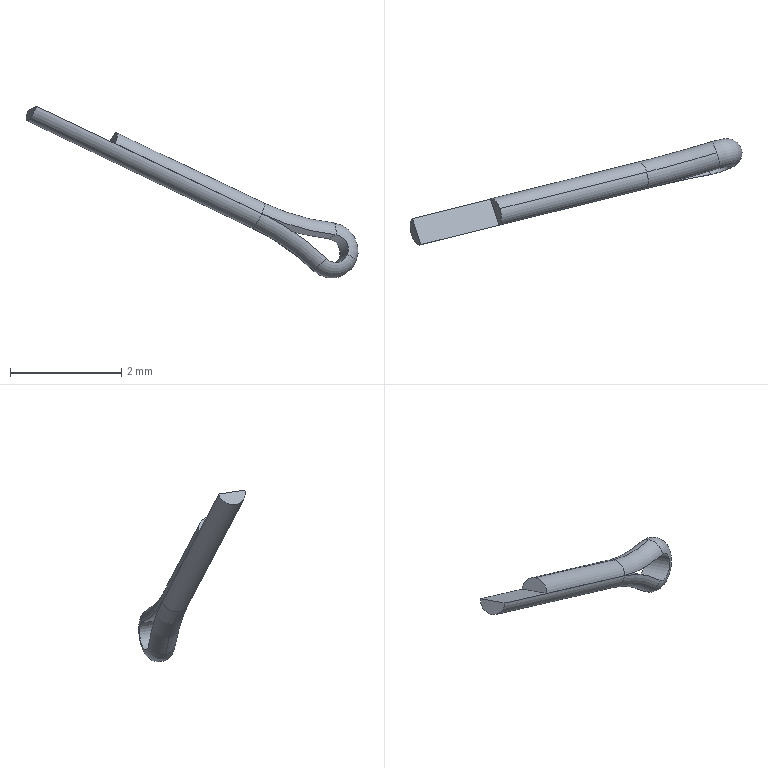Component | SolidWorks | split pins-2 | 1 solid | 16 faces | volume 1 mm3 | torus 6 | cylinder 6 | plane 4 | commonest cylinder face diameters 0.5 x4 8.75 x2
build123d program:
from build123d import *


with BuildPart() as part:
    # Body: sweep along a path in PathSke
    with BuildLine(Plane(origin=(1.208, 1.808, 0), x_dir=(0, 1, 0), z_dir=(0, 0, 1))) as body_path:
        Line((-1.558, -3.792), (-1.558, -0.792))
        ThreePointArc((-1.558, -0.792), (-1.502, -0.1139), (-1.335, 0.5458))
        ThreePointArc((-1.335, 0.5458), (-1.808, 1.208), (-2.281, 0.5458))
        ThreePointArc((-2.281, 0.5458), (-2.114, -0.1139), (-2.058, -0.792))
        Line((-2.058, -0.792), (-2.058, -5.392))
    # SectionSke → Body (sweep)
    with BuildSketch(Plane(origin=(5, 0.15, 0.15), x_dir=(0, 1, 0), z_dir=(1, 0, 0))):
        with BuildLine():
            Line((-0.15, -0.4), (-0.15, 0.1))
            ThreePointArc((-0.15, 0.1), (0.1, -0.15), (-0.15, -0.4))
        make_face()
    sweep(path=body_path.line)


solid = part.part

# Placed as in the assembly
solid = solid.moved(Location((-260.959, -17.55, 167.563), (-98.133, -17.491, -157.4)))
STEP:
#1=CARTESIAN_POINT('',(-10.34,-0.7059,6.639));
#2=VERTEX_POINT('',#1);
#3=CARTESIAN_POINT('',(-10.346,-0.699,6.629));
#4=VERTEX_POINT('',#3);
#5=CARTESIAN_POINT('',(-10.343,-0.7083,6.63));
#6=DIRECTION('',(-0.8805,-0.2203,0.4197));
#7=DIRECTION('',(0.3006,-0.9442,0.1349));
#8=AXIS2_PLACEMENT_3D('',#5,#6,#7);
#9=CIRCLE('',#8,0.009843);
#10=EDGE_CURVE('',#2,#4,#9,.T.);
#11=ORIENTED_EDGE('',*,*,#10,.F.);
#12=CARTESIAN_POINT('',(-10.29,-0.6921,6.625));
#13=VERTEX_POINT('',#12);
#14=CARTESIAN_POINT('',(-10.28,-0.6661,6.785));
#15=DIRECTION('',(0.3006,-0.9442,0.1349));
#16=DIRECTION('',(0.9529,0.3033,0.));
#17=AXIS2_PLACEMENT_3D('',#14,#15,#16);
#18=CIRCLE('',#17,0.1624);
#19=EDGE_CURVE('',#2,#13,#18,.T.);
#20=ORIENTED_EDGE('',*,*,#19,.T.);
#21=CARTESIAN_POINT('',(-10.294,-0.6844,6.614));
#22=VERTEX_POINT('',#21);
#23=CARTESIAN_POINT('',(-10.291,-0.6937,6.615));
#24=DIRECTION('',(-0.9518,-0.2879,0.1059));
#25=DIRECTION('',(0.3006,-0.9442,0.1349));
#26=AXIS2_PLACEMENT_3D('',#23,#24,#25);
#27=CIRCLE('',#26,0.009843);
#28=EDGE_CURVE('',#13,#22,#27,.T.);
#29=ORIENTED_EDGE('',*,*,#28,.T.);
#30=CARTESIAN_POINT('',(-10.283,-0.6568,6.783));
#31=DIRECTION('',(0.3006,-0.9442,0.1349));
#32=DIRECTION('',(0.8805,0.2203,-0.4197));
#33=AXIS2_PLACEMENT_3D('',#30,#31,#32);
#34=CIRCLE('',#33,0.1722);
#35=EDGE_CURVE('',#4,#22,#34,.T.);
#36=ORIENTED_EDGE('',*,*,#35,.F.);
#37=EDGE_LOOP('',(#11,#20,#29,#36));
#38=FACE_OUTER_BOUND('',#37,.T.);
#39=CARTESIAN_POINT('',(-10.28,-0.6661,6.785));
#40=DIRECTION('',(0.3006,-0.9442,0.1349));
#41=DIRECTION('',(0.8805,0.2203,-0.4197));
#42=AXIS2_PLACEMENT_3D('',#39,#40,#41);
#43=TOROIDAL_SURFACE('',#42,0.1722,0.009843);
#44=ADVANCED_FACE('',(#38),#43,.T.);
#45=CARTESIAN_POINT('',(-10.304,-0.7012,6.591));
#46=VERTEX_POINT('',#45);
#47=CARTESIAN_POINT('',(-10.3,-0.689,6.597));
#48=VERTEX_POINT('',#47);
#49=CARTESIAN_POINT('',(-10.298,-0.6983,6.598));
#50=DIRECTION('',(0.7141,0.129,-0.6881));
#51=DIRECTION('',(0.3006,-0.9442,0.1349));
#52=AXIS2_PLACEMENT_3D('',#49,#50,#51);
#53=CIRCLE('',#52,0.009843);
#54=EDGE_CURVE('',#46,#48,#53,.T.);
#55=ORIENTED_EDGE('',*,*,#54,.F.);
#56=CARTESIAN_POINT('',(-10.347,-0.7107,6.621));
#57=VERTEX_POINT('',#56);
#58=CARTESIAN_POINT('',(-10.406,-0.7505,6.475));
#59=DIRECTION('',(0.3006,-0.9442,0.1349));
#60=DIRECTION('',(0.9529,0.3033,0.));
#61=AXIS2_PLACEMENT_3D('',#58,#59,#60);
#62=CIRCLE('',#61,0.1624);
#63=EDGE_CURVE('',#46,#57,#62,.T.);
#64=ORIENTED_EDGE('',*,*,#63,.T.);
#65=CARTESIAN_POINT('',(-10.346,-0.699,6.629));
#66=VERTEX_POINT('',#65);
#67=CARTESIAN_POINT('',(-10.343,-0.7083,6.63));
#68=DIRECTION('',(0.8805,0.2203,-0.4197));
#69=DIRECTION('',(0.3006,-0.9442,0.1349));
#70=AXIS2_PLACEMENT_3D('',#67,#68,#69);
#71=CIRCLE('',#70,0.009843);
#72=EDGE_CURVE('',#57,#66,#71,.T.);
#73=ORIENTED_EDGE('',*,*,#72,.T.);
#74=CARTESIAN_POINT('',(-10.409,-0.7412,6.474));
#75=DIRECTION('',(0.3006,-0.9442,0.1349));
#76=DIRECTION('',(0.8805,0.2203,-0.4197));
#77=AXIS2_PLACEMENT_3D('',#74,#75,#76);
#78=CIRCLE('',#77,0.1722);
#79=EDGE_CURVE('',#48,#66,#78,.T.);
#80=ORIENTED_EDGE('',*,*,#79,.F.);
#81=EDGE_LOOP('',(#55,#64,#73,#80));
#82=FACE_OUTER_BOUND('',#81,.T.);
#83=CARTESIAN_POINT('',(-10.406,-0.7505,6.475));
#84=DIRECTION('',(0.3006,-0.9442,0.1349));
#85=DIRECTION('',(0.8805,0.2203,-0.4197));
#86=AXIS2_PLACEMENT_3D('',#83,#84,#85);
#87=TOROIDAL_SURFACE('',#86,0.1722,0.009843);
#88=ADVANCED_FACE('',(#82),#87,.T.);
#89=CARTESIAN_POINT('',(-10.34,-0.7176,6.631));
#90=VERTEX_POINT('',#89);
#91=CARTESIAN_POINT('',(-10.343,-0.7083,6.63));
#92=DIRECTION('',(-0.8805,-0.2203,0.4197));
#93=DIRECTION('',(0.3006,-0.9442,0.1349));
#94=AXIS2_PLACEMENT_3D('',#91,#92,#93);
#95=CIRCLE('',#94,0.009843);
#96=EDGE_CURVE('',#90,#2,#95,.T.);
#97=ORIENTED_EDGE('',*,*,#96,.T.);
#98=CARTESIAN_POINT('',(-10.444,-0.7319,6.688));
#99=VERTEX_POINT('',#98);
#100=CARTESIAN_POINT('',(-10.34,-0.7059,6.639));
#101=DIRECTION('',(-0.8805,-0.2203,0.4197));
#102=VECTOR('',#101,39.37);
#103=LINE('',#100,#102);
#104=EDGE_CURVE('',#2,#99,#103,.T.);
#105=ORIENTED_EDGE('',*,*,#104,.T.);
#106=CARTESIAN_POINT('',(-10.444,-0.7436,6.681));
#107=VERTEX_POINT('',#106);
#108=CARTESIAN_POINT('',(-10.447,-0.7343,6.68));
#109=DIRECTION('',(-0.8805,-0.2203,0.4197));
#110=DIRECTION('',(0.3006,-0.9442,0.1349));
#111=AXIS2_PLACEMENT_3D('',#108,#109,#110);
#112=CIRCLE('',#111,0.009843);
#113=EDGE_CURVE('',#107,#99,#112,.T.);
#114=ORIENTED_EDGE('',*,*,#113,.F.);
#115=CARTESIAN_POINT('',(-10.34,-0.7176,6.631));
#116=DIRECTION('',(-0.8805,-0.2203,0.4197));
#117=VECTOR('',#116,39.37);
#118=LINE('',#115,#117);
#119=EDGE_CURVE('',#90,#107,#118,.T.);
#120=ORIENTED_EDGE('',*,*,#119,.F.);
#121=EDGE_LOOP('',(#97,#105,#114,#120));
#122=FACE_OUTER_BOUND('',#121,.T.);
#123=CARTESIAN_POINT('',(-10.343,-0.7083,6.63));
#124=DIRECTION('',(-0.8805,-0.2203,0.4197));
#125=DIRECTION('',(0.3665,0.2449,0.8976));
#126=AXIS2_PLACEMENT_3D('',#123,#124,#125);
#127=CYLINDRICAL_SURFACE('',#126,0.009843);
#128=ADVANCED_FACE('',(#122),#127,.T.);
#129=CARTESIAN_POINT('',(-10.288,-0.703,6.616));
#130=VERTEX_POINT('',#129);
#131=CARTESIAN_POINT('',(-10.28,-0.7024,6.602));
#132=VERTEX_POINT('',#131);
#133=CARTESIAN_POINT('',(-10.288,-0.7046,6.607));
#134=DIRECTION('',(-0.3006,0.9442,-0.1349));
#135=DIRECTION('',(-0.8805,-0.2203,0.4197));
#136=AXIS2_PLACEMENT_3D('',#133,#134,#135);
#137=CIRCLE('',#136,0.009843);
#138=EDGE_CURVE('',#130,#132,#137,.T.);
#139=ORIENTED_EDGE('',*,*,#138,.T.);
#140=CARTESIAN_POINT('',(-10.286,-0.6838,6.6));
#141=VERTEX_POINT('',#140);
#142=CARTESIAN_POINT('',(-10.283,-0.6931,6.601));
#143=DIRECTION('',(0.3665,0.2449,0.8976));
#144=DIRECTION('',(0.9258,0.,-0.378));
#145=AXIS2_PLACEMENT_3D('',#142,#143,#144);
#146=CIRCLE('',#145,0.009843);
#147=EDGE_CURVE('',#132,#141,#146,.T.);
#148=ORIENTED_EDGE('',*,*,#147,.T.);
#149=CARTESIAN_POINT('',(-10.294,-0.686,6.604));
#150=DIRECTION('',(-0.3006,0.9442,-0.1349));
#151=DIRECTION('',(-0.8805,-0.2203,0.4197));
#152=AXIS2_PLACEMENT_3D('',#149,#150,#151);
#153=CIRCLE('',#152,0.009843);
#154=EDGE_CURVE('',#22,#141,#153,.T.);
#155=ORIENTED_EDGE('',*,*,#154,.F.);
#156=ORIENTED_EDGE('',*,*,#28,.F.);
#157=CARTESIAN_POINT('',(-10.291,-0.6937,6.615));
#158=DIRECTION('',(-0.9518,-0.2879,0.1059));
#159=DIRECTION('',(0.3006,-0.9442,0.1349));
#160=AXIS2_PLACEMENT_3D('',#157,#158,#159);
#161=CIRCLE('',#160,0.009843);
#162=EDGE_CURVE('',#130,#13,#161,.T.);
#163=ORIENTED_EDGE('',*,*,#162,.F.);
#164=EDGE_LOOP('',(#139,#148,#155,#156,#163));
#165=FACE_OUTER_BOUND('',#164,.T.);
#166=CARTESIAN_POINT('',(-10.291,-0.6953,6.605));
#167=DIRECTION('',(-0.3006,0.9442,-0.1349));
#168=DIRECTION('',(-0.8805,-0.2203,0.4197));
#169=AXIS2_PLACEMENT_3D('',#166,#167,#168);
#170=TOROIDAL_SURFACE('',#169,0.009843,0.009843);
#171=ADVANCED_FACE('',(#165),#170,.T.);
#172=CARTESIAN_POINT('',(-10.34,-0.7176,6.631));
#173=VERTEX_POINT('',#172);
#174=CARTESIAN_POINT('',(-10.34,-0.7176,6.631));
#175=DIRECTION('',(0.3006,-0.9442,0.1349));
#176=VECTOR('',#175,39.37);
#177=LINE('',#174,#176);
#178=EDGE_CURVE('',#66,#173,#177,.T.);
#179=ORIENTED_EDGE('',*,*,#178,.F.);
#180=CARTESIAN_POINT('',(-10.506,-0.7389,6.705));
#181=VERTEX_POINT('',#180);
#182=CARTESIAN_POINT('',(-10.346,-0.699,6.629));
#183=DIRECTION('',(-0.8805,-0.2203,0.4197));
#184=VECTOR('',#183,39.37);
#185=LINE('',#182,#184);
#186=EDGE_CURVE('',#66,#181,#185,.T.);
#187=ORIENTED_EDGE('',*,*,#186,.T.);
#188=CARTESIAN_POINT('',(-10.5,-0.7575,6.707));
#189=VERTEX_POINT('',#188);
#190=CARTESIAN_POINT('',(-10.5,-0.7575,6.707));
#191=DIRECTION('',(0.3006,-0.9442,0.1349));
#192=VECTOR('',#191,39.37);
#193=LINE('',#190,#192);
#194=EDGE_CURVE('',#181,#189,#193,.T.);
#195=ORIENTED_EDGE('',*,*,#194,.T.);
#196=CARTESIAN_POINT('',(-10.34,-0.7176,6.631));
#197=DIRECTION('',(-0.8805,-0.2203,0.4197));
#198=VECTOR('',#197,39.37);
#199=LINE('',#196,#198);
#200=EDGE_CURVE('',#173,#189,#199,.T.);
#201=ORIENTED_EDGE('',*,*,#200,.F.);
#202=EDGE_LOOP('',(#179,#187,#195,#201));
#203=FACE_OUTER_BOUND('',#202,.T.);
#204=CARTESIAN_POINT('',(-10.34,-0.7176,6.631));
#205=DIRECTION('',(-0.3665,-0.2449,-0.8976));
#206=DIRECTION('',(-0.8805,-0.2203,0.4197));
#207=AXIS2_PLACEMENT_3D('',#204,#205,#206);
#208=PLANE('',#207);
#209=ADVANCED_FACE('',(#203),#208,.F.);
#210=CARTESIAN_POINT('',(-10.343,-0.7083,6.63));
#211=DIRECTION('',(0.8805,0.2203,-0.4197));
#212=DIRECTION('',(0.3006,-0.9442,0.1349));
#213=AXIS2_PLACEMENT_3D('',#210,#211,#212);
#214=CIRCLE('',#213,0.009843);
#215=EDGE_CURVE('',#173,#57,#214,.T.);
#216=ORIENTED_EDGE('',*,*,#215,.F.);
#217=ORIENTED_EDGE('',*,*,#200,.T.);
#218=CARTESIAN_POINT('',(-10.503,-0.7482,6.706));
#219=DIRECTION('',(0.8805,0.2203,-0.4197));
#220=DIRECTION('',(0.3006,-0.9442,0.1349));
#221=AXIS2_PLACEMENT_3D('',#218,#219,#220);
#222=CIRCLE('',#221,0.009843);
#223=EDGE_CURVE('',#189,#181,#222,.T.);
#224=ORIENTED_EDGE('',*,*,#223,.T.);
#225=ORIENTED_EDGE('',*,*,#186,.F.);
#226=ORIENTED_EDGE('',*,*,#72,.F.);
#227=EDGE_LOOP('',(#216,#217,#224,#225,#226));
#228=FACE_OUTER_BOUND('',#227,.T.);
#229=CARTESIAN_POINT('',(-10.343,-0.7083,6.63));
#230=DIRECTION('',(-0.8805,-0.2203,0.4197));
#231=DIRECTION('',(0.3665,0.2449,0.8976));
#232=AXIS2_PLACEMENT_3D('',#229,#230,#231);
#233=CYLINDRICAL_SURFACE('',#232,0.009843);
#234=ADVANCED_FACE('',(#228),#233,.T.);
#235=CARTESIAN_POINT('',(-10.295,-0.7075,6.6));
#236=VERTEX_POINT('',#235);
#237=CARTESIAN_POINT('',(-10.295,-0.7075,6.6));
#238=DIRECTION('',(0.3006,-0.9442,0.1349));
#239=VECTOR('',#238,39.37);
#240=LINE('',#237,#239);
#241=EDGE_CURVE('',#48,#236,#240,.T.);
#242=ORIENTED_EDGE('',*,*,#241,.F.);
#243=ORIENTED_EDGE('',*,*,#79,.T.);
#244=ORIENTED_EDGE('',*,*,#178,.T.);
#245=CARTESIAN_POINT('',(-10.403,-0.7598,6.477));
#246=DIRECTION('',(0.3006,-0.9442,0.1349));
#247=DIRECTION('',(0.8805,0.2203,-0.4197));
#248=AXIS2_PLACEMENT_3D('',#245,#246,#247);
#249=CIRCLE('',#248,0.1722);
#250=EDGE_CURVE('',#236,#173,#249,.T.);
#251=ORIENTED_EDGE('',*,*,#250,.F.);
#252=EDGE_LOOP('',(#242,#243,#244,#251));
#253=FACE_OUTER_BOUND('',#252,.T.);
#254=CARTESIAN_POINT('',(-10.406,-0.7505,6.475));
#255=DIRECTION('',(0.3006,-0.9442,0.1349));
#256=DIRECTION('',(0.8805,0.2203,-0.4197));
#257=AXIS2_PLACEMENT_3D('',#254,#255,#256);
#258=CYLINDRICAL_SURFACE('',#257,0.1722);
#259=ADVANCED_FACE('',(#253),#258,.T.);
#260=ORIENTED_EDGE('',*,*,#63,.F.);
#261=CARTESIAN_POINT('',(-10.298,-0.6983,6.598));
#262=DIRECTION('',(0.7141,0.129,-0.6881));
#263=DIRECTION('',(0.3006,-0.9442,0.1349));
#264=AXIS2_PLACEMENT_3D('',#261,#262,#263);
#265=CIRCLE('',#264,0.009843);
#266=EDGE_CURVE('',#236,#46,#265,.T.);
#267=ORIENTED_EDGE('',*,*,#266,.F.);
#268=ORIENTED_EDGE('',*,*,#250,.T.);
#269=ORIENTED_EDGE('',*,*,#215,.T.);
#270=EDGE_LOOP('',(#260,#267,#268,#269));
#271=FACE_OUTER_BOUND('',#270,.T.);
#272=CARTESIAN_POINT('',(-10.406,-0.7505,6.475));
#273=DIRECTION('',(0.3006,-0.9442,0.1349));
#274=DIRECTION('',(0.8805,0.2203,-0.4197));
#275=AXIS2_PLACEMENT_3D('',#272,#273,#274);
#276=TOROIDAL_SURFACE('',#275,0.1722,0.009843);
#277=ADVANCED_FACE('',(#271),#276,.T.);
#278=CARTESIAN_POINT('',(-10.288,-0.703,6.616));
#279=DIRECTION('',(0.3006,-0.9442,0.1349));
#280=VECTOR('',#279,39.37);
#281=LINE('',#278,#280);
#282=EDGE_CURVE('',#22,#130,#281,.T.);
#283=ORIENTED_EDGE('',*,*,#282,.F.);
#284=ORIENTED_EDGE('',*,*,#154,.T.);
#285=CARTESIAN_POINT('',(-10.294,-0.686,6.604));
#286=DIRECTION('',(-0.3006,0.9442,-0.1349));
#287=DIRECTION('',(-0.8805,-0.2203,0.4197));
#288=AXIS2_PLACEMENT_3D('',#285,#286,#287);
#289=CIRCLE('',#288,0.009843);
#290=EDGE_CURVE('',#141,#48,#289,.T.);
#291=ORIENTED_EDGE('',*,*,#290,.T.);
#292=ORIENTED_EDGE('',*,*,#241,.T.);
#293=CARTESIAN_POINT('',(-10.288,-0.7046,6.607));
#294=DIRECTION('',(-0.3006,0.9442,-0.1349));
#295=DIRECTION('',(-0.8805,-0.2203,0.4197));
#296=AXIS2_PLACEMENT_3D('',#293,#294,#295);
#297=CIRCLE('',#296,0.009843);
#298=EDGE_CURVE('',#132,#236,#297,.T.);
#299=ORIENTED_EDGE('',*,*,#298,.F.);
#300=ORIENTED_EDGE('',*,*,#138,.F.);
#301=EDGE_LOOP('',(#283,#284,#291,#292,#299,#300));
#302=FACE_OUTER_BOUND('',#301,.T.);
#303=CARTESIAN_POINT('',(-10.291,-0.6953,6.605));
#304=DIRECTION('',(-0.3006,0.9442,-0.1349));
#305=DIRECTION('',(-0.8805,-0.2203,0.4197));
#306=AXIS2_PLACEMENT_3D('',#303,#304,#305);
#307=CYLINDRICAL_SURFACE('',#306,0.009843);
#308=ADVANCED_FACE('',(#302),#307,.F.);
#309=ORIENTED_EDGE('',*,*,#147,.F.);
#310=ORIENTED_EDGE('',*,*,#298,.T.);
#311=ORIENTED_EDGE('',*,*,#266,.T.);
#312=ORIENTED_EDGE('',*,*,#54,.T.);
#313=ORIENTED_EDGE('',*,*,#290,.F.);
#314=EDGE_LOOP('',(#309,#310,#311,#312,#313));
#315=FACE_OUTER_BOUND('',#314,.T.);
#316=CARTESIAN_POINT('',(-10.291,-0.6953,6.605));
#317=DIRECTION('',(-0.3006,0.9442,-0.1349));
#318=DIRECTION('',(-0.8805,-0.2203,0.4197));
#319=AXIS2_PLACEMENT_3D('',#316,#317,#318);
#320=TOROIDAL_SURFACE('',#319,0.009843,0.009843);
#321=ADVANCED_FACE('',(#315),#320,.T.);
#322=CARTESIAN_POINT('',(-10.34,-0.7176,6.631));
#323=DIRECTION('',(0.3006,-0.9442,0.1349));
#324=VECTOR('',#323,39.37);
#325=LINE('',#322,#324);
#326=EDGE_CURVE('',#4,#90,#325,.T.);
#327=ORIENTED_EDGE('',*,*,#326,.F.);
#328=ORIENTED_EDGE('',*,*,#35,.T.);
#329=ORIENTED_EDGE('',*,*,#282,.T.);
#330=CARTESIAN_POINT('',(-10.277,-0.6754,6.786));
#331=DIRECTION('',(0.3006,-0.9442,0.1349));
#332=DIRECTION('',(0.8805,0.2203,-0.4197));
#333=AXIS2_PLACEMENT_3D('',#330,#331,#332);
#334=CIRCLE('',#333,0.1722);
#335=EDGE_CURVE('',#90,#130,#334,.T.);
#336=ORIENTED_EDGE('',*,*,#335,.F.);
#337=EDGE_LOOP('',(#327,#328,#329,#336));
#338=FACE_OUTER_BOUND('',#337,.T.);
#339=CARTESIAN_POINT('',(-10.28,-0.6661,6.785));
#340=DIRECTION('',(0.3006,-0.9442,0.1349));
#341=DIRECTION('',(0.8805,0.2203,-0.4197));
#342=AXIS2_PLACEMENT_3D('',#339,#340,#341);
#343=CYLINDRICAL_SURFACE('',#342,0.1722);
#344=ADVANCED_FACE('',(#338),#343,.T.);
#345=ORIENTED_EDGE('',*,*,#19,.F.);
#346=ORIENTED_EDGE('',*,*,#96,.F.);
#347=ORIENTED_EDGE('',*,*,#335,.T.);
#348=ORIENTED_EDGE('',*,*,#162,.T.);
#349=EDGE_LOOP('',(#345,#346,#347,#348));
#350=FACE_OUTER_BOUND('',#349,.T.);
#351=CARTESIAN_POINT('',(-10.28,-0.6661,6.785));
#352=DIRECTION('',(0.3006,-0.9442,0.1349));
#353=DIRECTION('',(0.8805,0.2203,-0.4197));
#354=AXIS2_PLACEMENT_3D('',#351,#352,#353);
#355=TOROIDAL_SURFACE('',#354,0.1722,0.009843);
#356=ADVANCED_FACE('',(#350),#355,.T.);
#357=ORIENTED_EDGE('',*,*,#104,.F.);
#358=ORIENTED_EDGE('',*,*,#10,.T.);
#359=CARTESIAN_POINT('',(-10.45,-0.725,6.678));
#360=VERTEX_POINT('',#359);
#361=CARTESIAN_POINT('',(-10.346,-0.699,6.629));
#362=DIRECTION('',(-0.8805,-0.2203,0.4197));
#363=VECTOR('',#362,39.37);
#364=LINE('',#361,#363);
#365=EDGE_CURVE('',#4,#360,#364,.T.);
#366=ORIENTED_EDGE('',*,*,#365,.T.);
#367=CARTESIAN_POINT('',(-10.447,-0.7343,6.68));
#368=DIRECTION('',(-0.8805,-0.2203,0.4197));
#369=DIRECTION('',(0.3006,-0.9442,0.1349));
#370=AXIS2_PLACEMENT_3D('',#367,#368,#369);
#371=CIRCLE('',#370,0.009843);
#372=EDGE_CURVE('',#99,#360,#371,.T.);
#373=ORIENTED_EDGE('',*,*,#372,.F.);
#374=EDGE_LOOP('',(#357,#358,#366,#373));
#375=FACE_OUTER_BOUND('',#374,.T.);
#376=CARTESIAN_POINT('',(-10.343,-0.7083,6.63));
#377=DIRECTION('',(-0.8805,-0.2203,0.4197));
#378=DIRECTION('',(0.3665,0.2449,0.8976));
#379=AXIS2_PLACEMENT_3D('',#376,#377,#378);
#380=CYLINDRICAL_SURFACE('',#379,0.009843);
#381=ADVANCED_FACE('',(#375),#380,.T.);
#382=CARTESIAN_POINT('',(-10.444,-0.7436,6.681));
#383=DIRECTION('',(0.3006,-0.9442,0.1349));
#384=VECTOR('',#383,39.37);
#385=LINE('',#382,#384);
#386=EDGE_CURVE('',#360,#107,#385,.T.);
#387=ORIENTED_EDGE('',*,*,#386,.F.);
#388=ORIENTED_EDGE('',*,*,#365,.F.);
#389=ORIENTED_EDGE('',*,*,#326,.T.);
#390=ORIENTED_EDGE('',*,*,#119,.T.);
#391=EDGE_LOOP('',(#387,#388,#389,#390));
#392=FACE_OUTER_BOUND('',#391,.T.);
#393=CARTESIAN_POINT('',(-10.34,-0.7176,6.631));
#394=DIRECTION('',(-0.3665,-0.2449,-0.8976));
#395=DIRECTION('',(-0.8805,-0.2203,0.4197));
#396=AXIS2_PLACEMENT_3D('',#393,#394,#395);
#397=PLANE('',#396);
#398=ADVANCED_FACE('',(#392),#397,.T.);
#399=ORIENTED_EDGE('',*,*,#223,.F.);
#400=ORIENTED_EDGE('',*,*,#194,.F.);
#401=EDGE_LOOP('',(#399,#400));
#402=FACE_OUTER_BOUND('',#401,.T.);
#403=CARTESIAN_POINT('',(-10.503,-0.7482,6.706));
#404=DIRECTION('',(0.8805,0.2203,-0.4197));
#405=DIRECTION('',(0.3006,-0.9442,0.1349));
#406=AXIS2_PLACEMENT_3D('',#403,#404,#405);
#407=PLANE('',#406);
#408=ADVANCED_FACE('',(#402),#407,.F.);
#409=ORIENTED_EDGE('',*,*,#113,.T.);
#410=ORIENTED_EDGE('',*,*,#372,.T.);
#411=ORIENTED_EDGE('',*,*,#386,.T.);
#412=EDGE_LOOP('',(#409,#410,#411));
#413=FACE_OUTER_BOUND('',#412,.T.);
#414=CARTESIAN_POINT('',(-10.447,-0.7343,6.68));
#415=DIRECTION('',(-0.8805,-0.2203,0.4197));
#416=DIRECTION('',(0.3006,-0.9442,0.1349));
#417=AXIS2_PLACEMENT_3D('',#414,#415,#416);
#418=PLANE('',#417);
#419=ADVANCED_FACE('',(#413),#418,.T.);
#420=CLOSED_SHELL('',(#44,#88,#128,#171,#209,#234,#259,#277,#308,#321,#344,#356,#381,#398,#408,#419));
#421=MANIFOLD_SOLID_BREP('',#420);
#422=CARTESIAN_POINT('',(0.,0.,0.));
#423=DIRECTION('',(0.,0.,1.));
#424=DIRECTION('',(1.,0.,0.));
#425=AXIS2_PLACEMENT_3D('',#422,#423,#424);
#426=(LENGTH_UNIT()NAMED_UNIT(*)SI_UNIT($,.METRE.));
#427=LENGTH_MEASURE_WITH_UNIT(LENGTH_MEASURE(0.0254),#426);
#428=DIMENSIONAL_EXPONENTS(1.,0.,0.,0.,0.,0.,0.);
#429=(CONVERSION_BASED_UNIT('',#427)LENGTH_UNIT()NAMED_UNIT(#428));
#430=UNCERTAINTY_MEASURE_WITH_UNIT(LENGTH_MEASURE(0.00001),#429,'','');
#431=(NAMED_UNIT(*)PLANE_ANGLE_UNIT()SI_UNIT($,.RADIAN.));
#432=(NAMED_UNIT(*)SI_UNIT($,.STERADIAN.)SOLID_ANGLE_UNIT());
#433=(GEOMETRIC_REPRESENTATION_CONTEXT(3)GLOBAL_UNCERTAINTY_ASSIGNED_CONTEXT((#430))GLOBAL_UNIT_ASSIGNED_CONTEXT((#429,#431,#432))REPRESENTATION_CONTEXT('',''));
#434=ADVANCED_BREP_SHAPE_REPRESENTATION('',(#421,#425),#433);
#435=COLOUR_RGB('',0.7922,0.8196,0.9333);
#436=FILL_AREA_STYLE_COLOUR('',#435);
#437=FILL_AREA_STYLE('',(#436));
#438=SURFACE_STYLE_FILL_AREA(#437);
#439=SURFACE_SIDE_STYLE('',(#438));
#440=SURFACE_STYLE_USAGE(.BOTH.,#439);
#441=PRESENTATION_STYLE_ASSIGNMENT((#440));
#442=STYLED_ITEM('',(#441),#421);
#443=PRESENTATION_LAYER_ASSIGNMENT('','',(#442));
#444=(LENGTH_UNIT()NAMED_UNIT(*)SI_UNIT($,.METRE.));
#445=LENGTH_MEASURE_WITH_UNIT(LENGTH_MEASURE(0.0254),#444);
#446=DIMENSIONAL_EXPONENTS(1.,0.,0.,0.,0.,0.,0.);
#447=(CONVERSION_BASED_UNIT('',#445)LENGTH_UNIT()NAMED_UNIT(#446));
#448=UNCERTAINTY_MEASURE_WITH_UNIT(LENGTH_MEASURE(0.00001),#447,'','');
#449=(NAMED_UNIT(*)PLANE_ANGLE_UNIT()SI_UNIT($,.RADIAN.));
#450=(NAMED_UNIT(*)SI_UNIT($,.STERADIAN.)SOLID_ANGLE_UNIT());
#451=(GEOMETRIC_REPRESENTATION_CONTEXT(3)GLOBAL_UNCERTAINTY_ASSIGNED_CONTEXT((#448))GLOBAL_UNIT_ASSIGNED_CONTEXT((#447,#449,#450))REPRESENTATION_CONTEXT('',''));
#452=MECHANICAL_DESIGN_GEOMETRIC_PRESENTATION_REPRESENTATION('',(#442),#451);